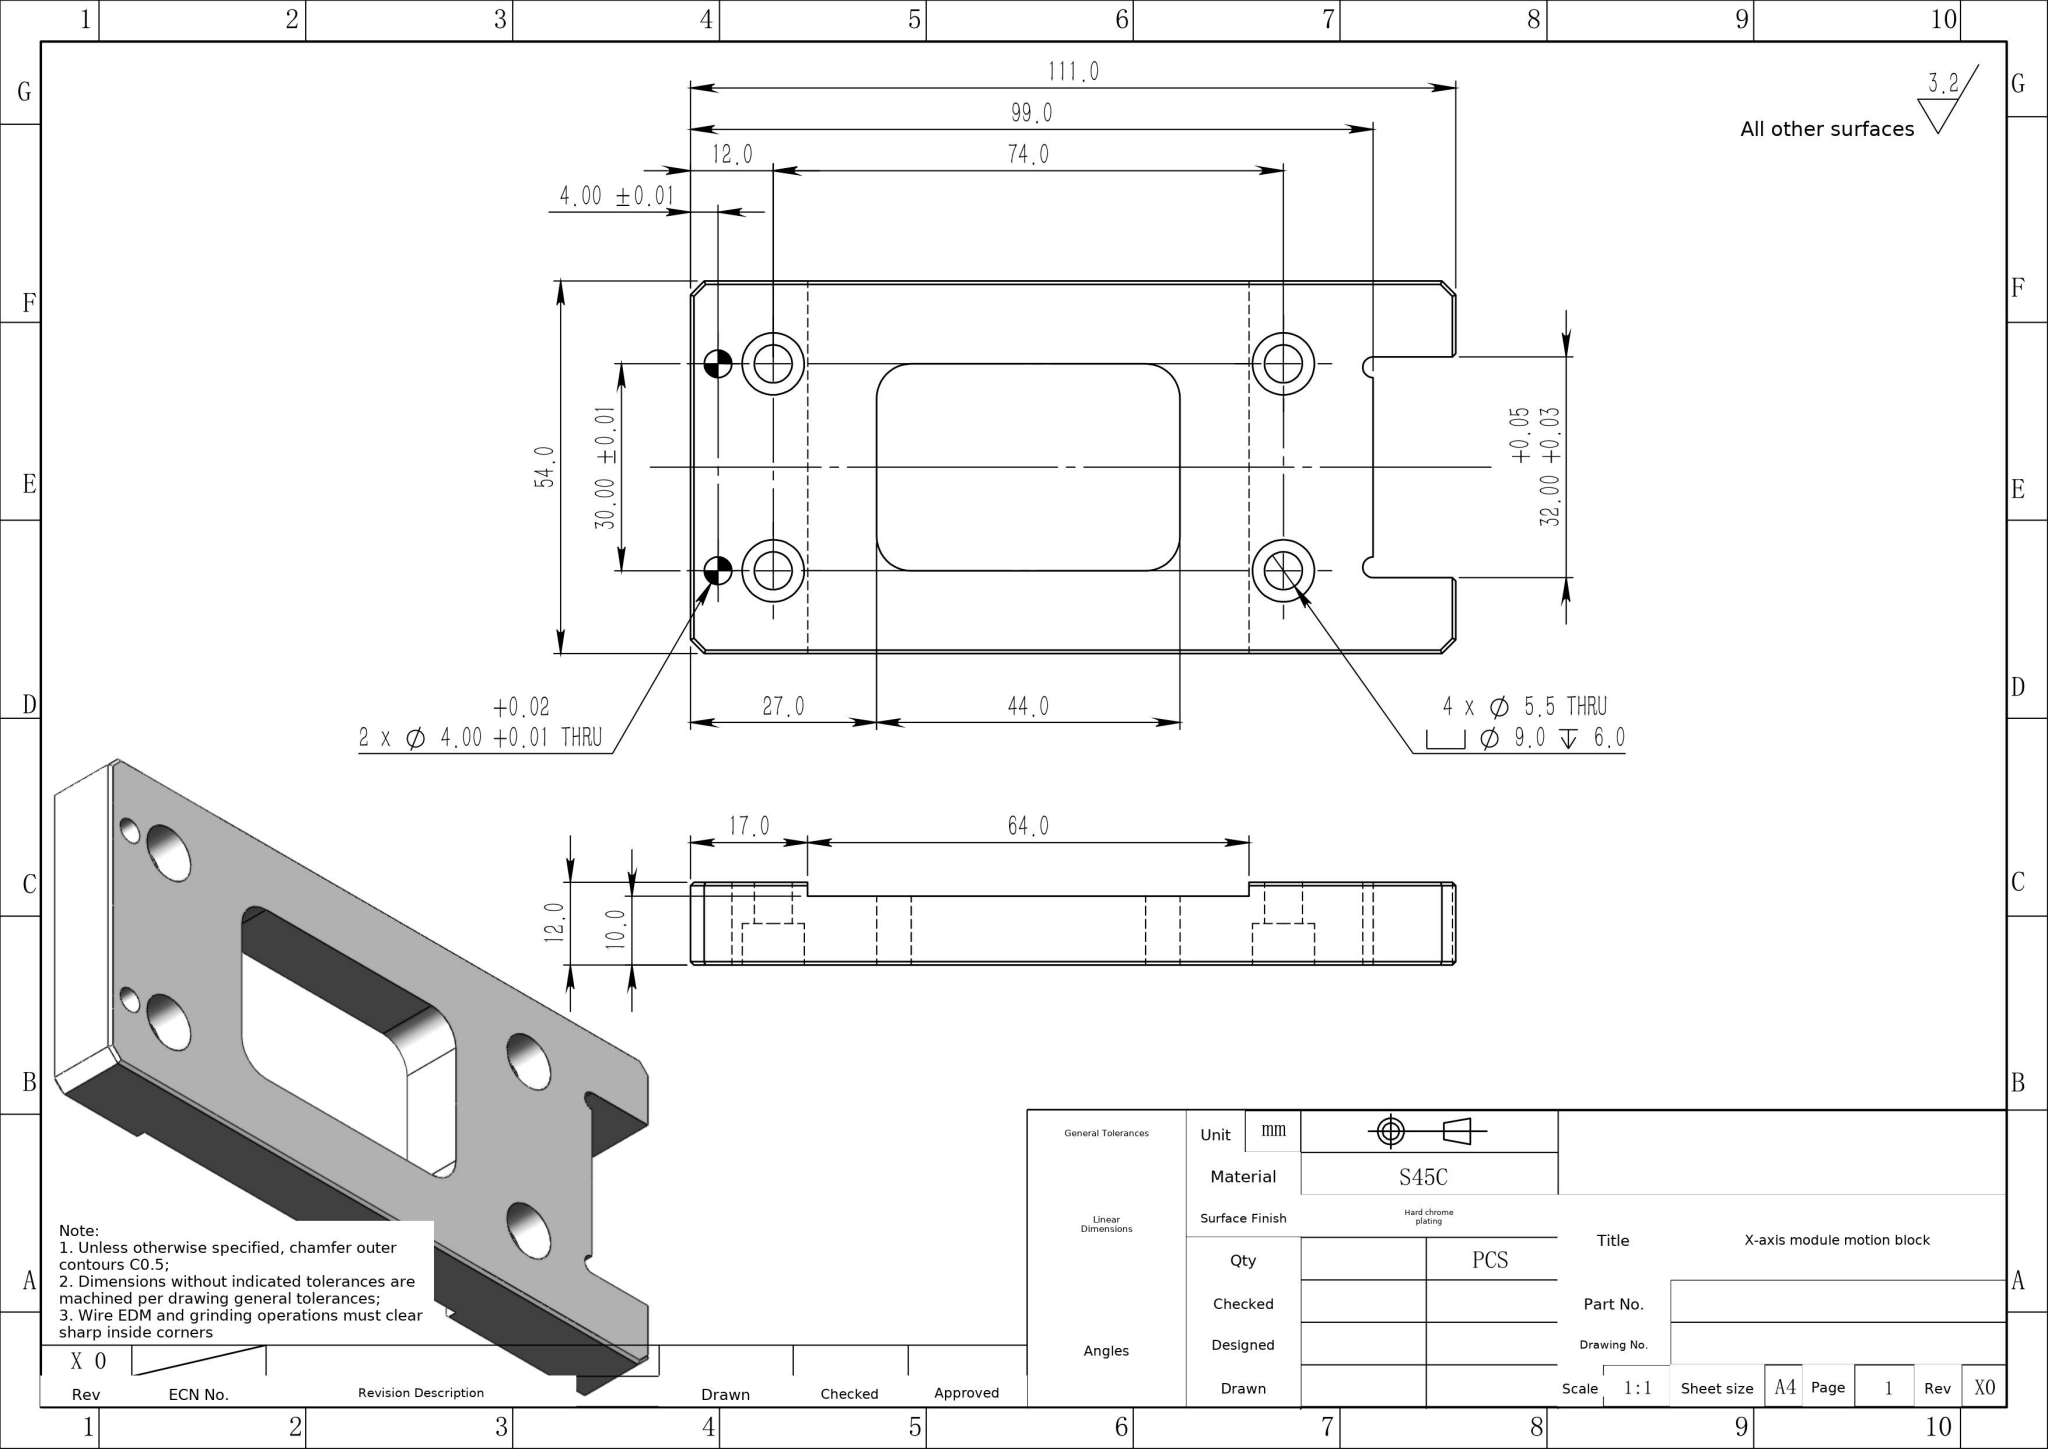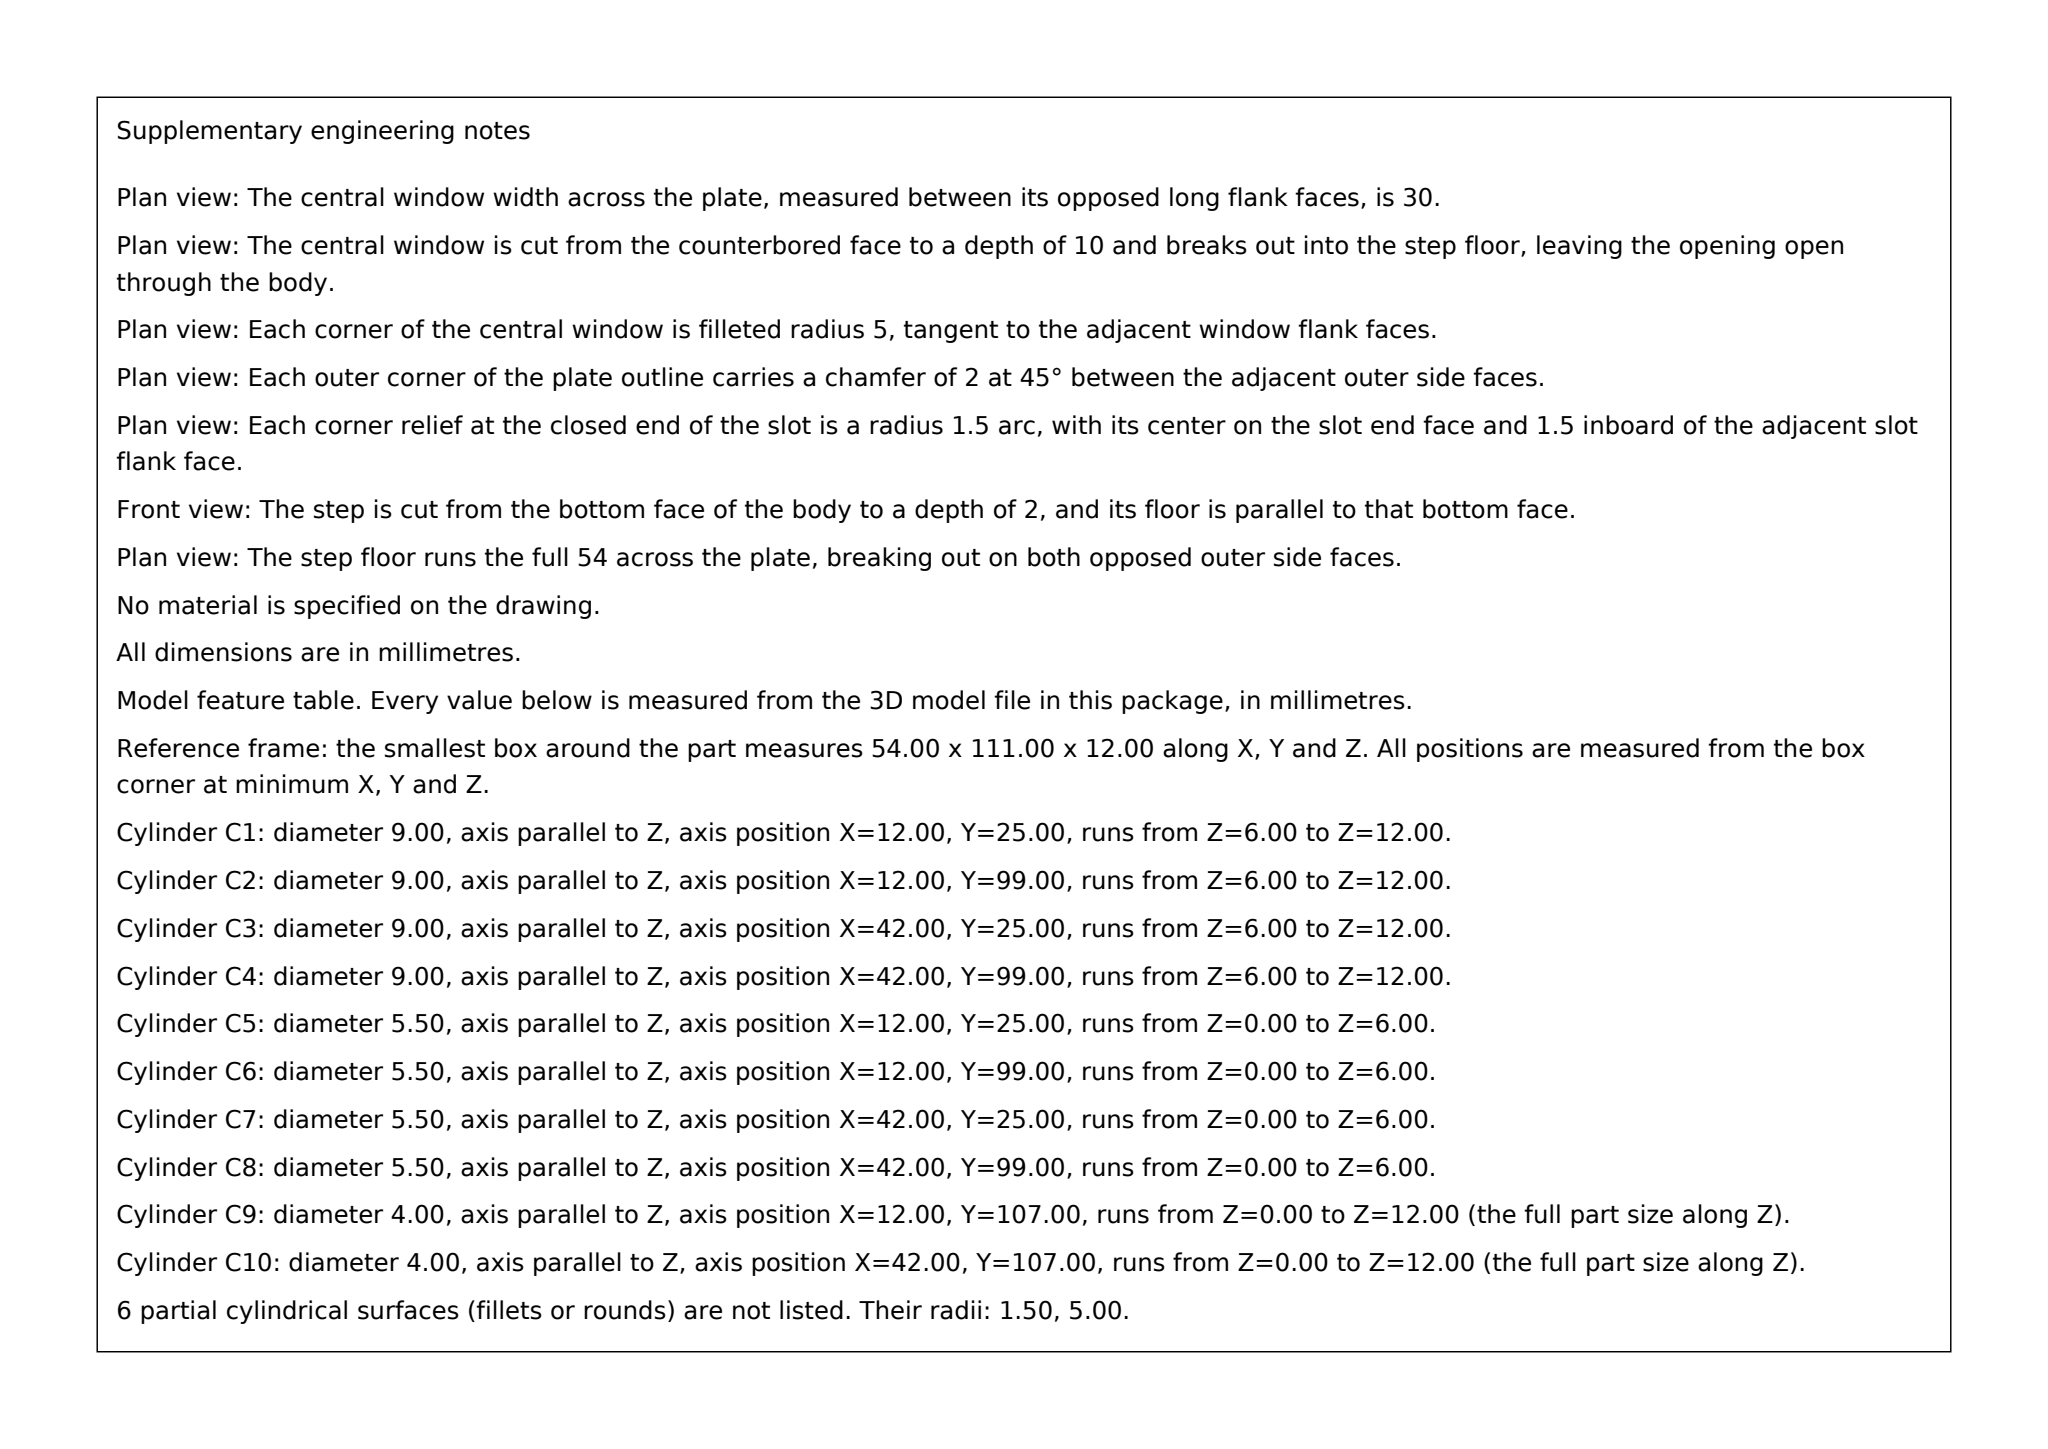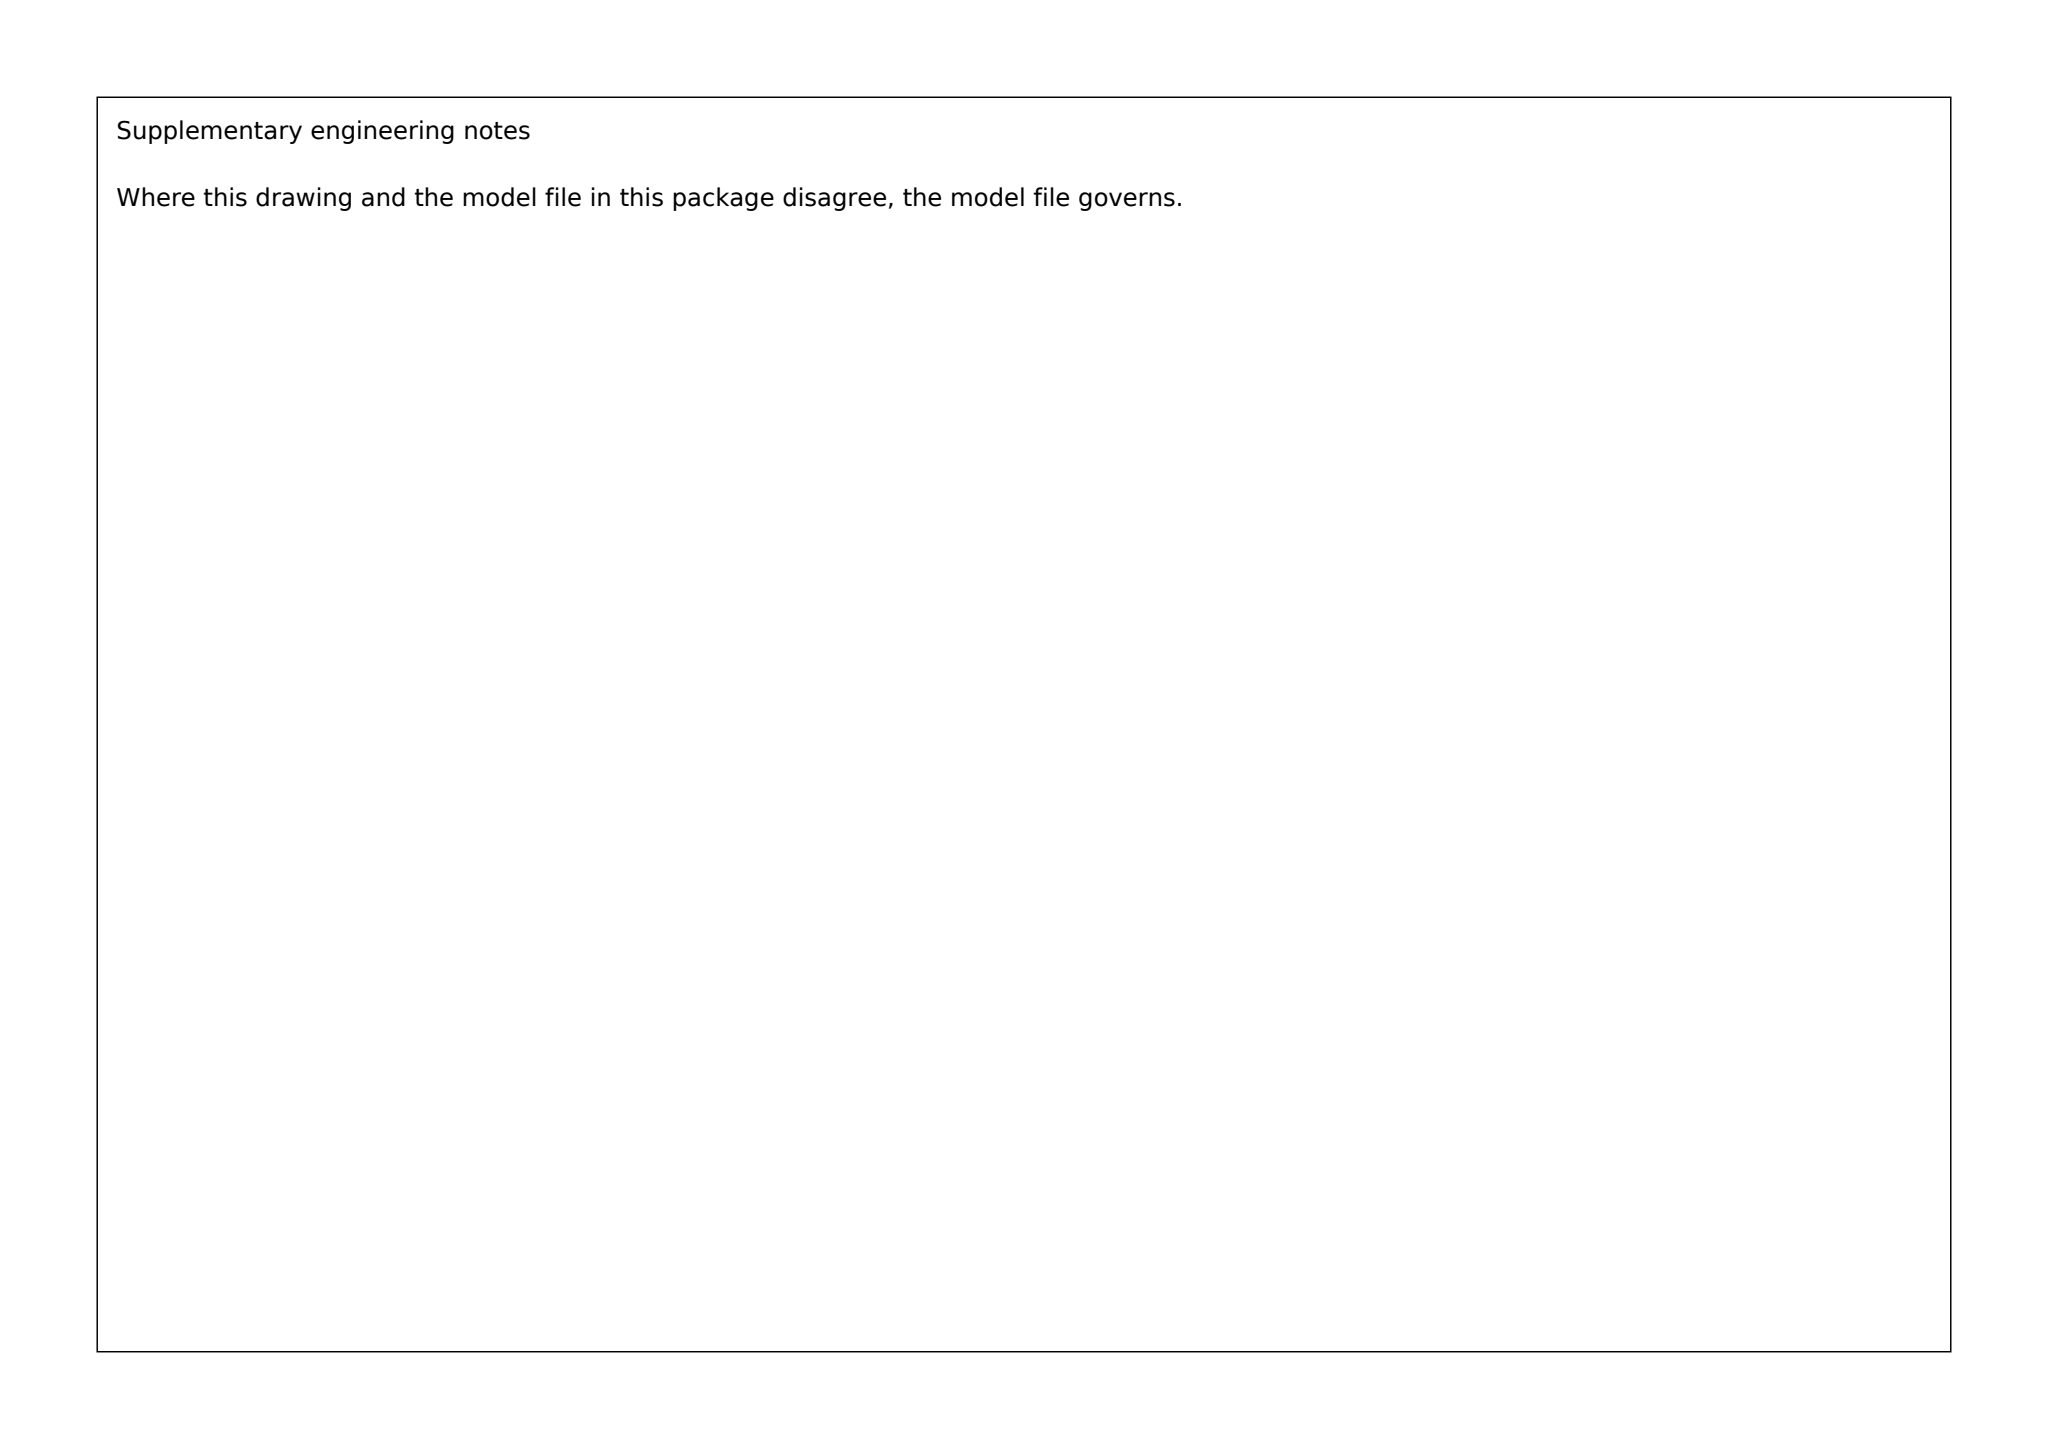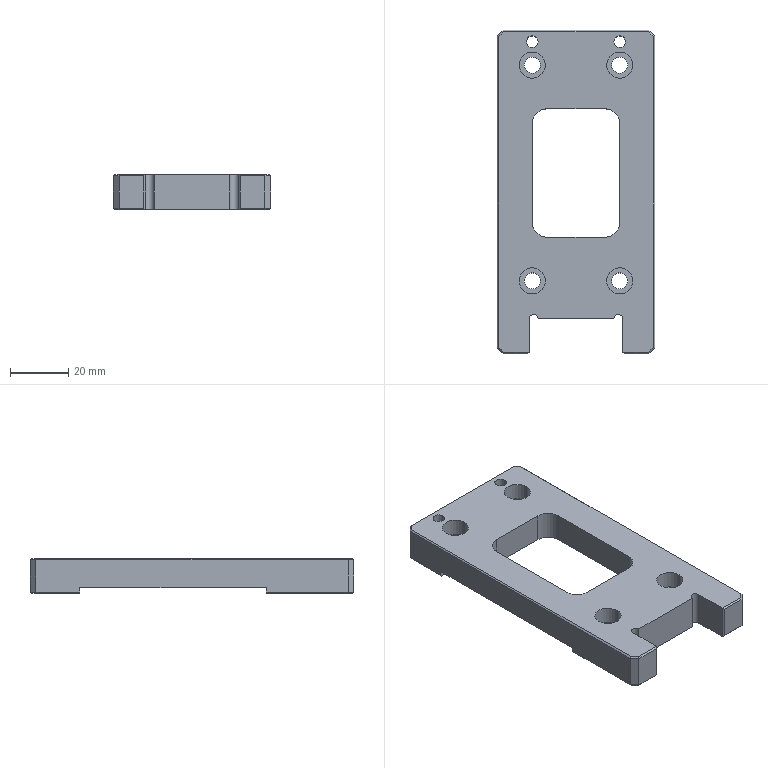Part | SolidWorks | mm | 1 solid | 74 faces | box 54 x 111 x 12 mm | volume 44783 mm3 | plane 48 | cylinder 26 | commonest cylinder face diameters 9 x8 5.5 x8 4 x4 10 x4 3 x2
build123d program:
from build123d import *

# Parameters (mm, degrees)
SKETCH1_W                                       = 54
SKETCH1_H                                       = 111
BOSS_EXTRUDE1_DEPTH                             = 12
M5_HEX_SOCKET_HEAD_CAP_SCREW_CBORE1_D           = 5.5
M5_HEX_SOCKET_HEAD_CAP_SCREW_CBORE1_CBORE_D     = 9
M5_HEX_SOCKET_HEAD_CAP_SCREW_CBORE1_CBORE_DEPTH = 6
SKETCH5_W                                       = 32
SKETCH5_H                                       = 12
CUT_EXTRUDE2_DEPTH                              = 63.875
SIZE_MM_DOWEL_PIN_HOLE1_D                       = 4
SKETCH8_R                                       = 1.5
CUT_EXTRUDE3_DEPTH                              = 63.875
SKETCH9_W                                       = 54
SKETCH9_H                                       = 64
CUT_EXTRUDE4_DEPTH                              = 2
SKETCH11_W                                      = 30
SKETCH11_H                                      = 44
CUT_EXTRUDE5_DEPTH                              = 63.524
CHAMFER1_SIZE                                   = 2
CHAMFER2_SIZE                                   = 0.5
FILLET1_R                                       = 5


with BuildPart() as part:
    # Sketch1 → Boss-Extrude1 (new body)
    with BuildSketch(Plane.XY):
        Rectangle(SKETCH1_W, SKETCH1_H)
    extrude(amount=-BOSS_EXTRUDE1_DEPTH)

    # M5 Hex Socket Head Cap Screw CBORE1 (through all)
    with Locations(Plane.XY):
        with Locations((-15, -30.5), (-15, 43.5), (15, 43.5), (15, -30.5)):
            CounterBoreHole(M5_HEX_SOCKET_HEAD_CAP_SCREW_CBORE1_D / 2, M5_HEX_SOCKET_HEAD_CAP_SCREW_CBORE1_CBORE_D / 2, M5_HEX_SOCKET_HEAD_CAP_SCREW_CBORE1_CBORE_DEPTH)

    # Sketch5 → Cut-Extrude2 (cut, through all)
    with BuildSketch(Plane.XY):
        with Locations((0, -49.5)):
            Rectangle(SKETCH5_W, SKETCH5_H)
    extrude(amount=-CUT_EXTRUDE2_DEPTH, mode=Mode.SUBTRACT)

    # Size mm Dowel Pin Hole1 (through all)
    with Locations(Plane.XY):
        with Locations((-15, 51.5), (15, 51.5)):
            Hole(SIZE_MM_DOWEL_PIN_HOLE1_D / 2)

    # Sketch8 → Cut-Extrude3 (cut, through all)
    with BuildSketch(Plane.XY):
        with Locations((-14.5, -43.5)):
            Circle(SKETCH8_R)
        with Locations((14.5, -43.5)):
            Circle(SKETCH8_R)
    extrude(amount=-CUT_EXTRUDE3_DEPTH, mode=Mode.SUBTRACT)

    # Sketch9 → Cut-Extrude4 (cut)
    with BuildSketch(Plane(origin=(0, 0, -12), x_dir=(-1, 0, 0), z_dir=(0, 0, -1))):
        with Locations((0, 6.5)):
            Rectangle(SKETCH9_W, SKETCH9_H)
    extrude(amount=-CUT_EXTRUDE4_DEPTH, mode=Mode.SUBTRACT)

    # Sketch11 → Cut-Extrude5 (cut, through all)
    with BuildSketch(Plane(origin=(0, 0, -10), x_dir=(-1, 0, 0), z_dir=(0, 0, -1))):
        with Locations((0, 6.5)):
            Rectangle(SKETCH11_W, SKETCH11_H)
    extrude(amount=-CUT_EXTRUDE5_DEPTH, mode=Mode.SUBTRACT)

    # Chamfer1
    chamfer1_edges = [part.edges().sort_by_distance(p)[0] for p in [
        (27, -55.5, -6),
        (-27, -55.5, -6),
        (-27, 55.5, -6),
        (27, 55.5, -6),
    ]]
    chamfer(chamfer1_edges, length=CHAMFER1_SIZE)

    # Chamfer2
    chamfer2_edges = [part.edges().sort_by_distance(p)[0] for p in [
        (27, 0, 0),
        (27, -39.5, -12),
        (0, 55.5, 0),
        (-27, 0, 0),
        (-20.5, -55.5, 0),
        (26, -54.5, 0),
        (-26, -54.5, 0),
        (-26, 54.5, 0),
        (26, 54.5, 0),
        (0, 55.5, -12),
        (-27, 46, -12),
        (-26, 54.5, -12),
        (26, 54.5, -12),
        (-20.5, -55.5, -12),
        (26, -54.5, -12),
        (-26, -54.5, -12),
        (20.5, -55.5, 0),
        (20.5, -55.5, -12),
        (-16, -55.5, -6),
        (16, -55.5, -6),
        (-27, -39.5, -12),
        (27, 46, -12),
    ]]
    chamfer(chamfer2_edges, length=CHAMFER2_SIZE)

    # Fillet1
    fillet1_edges = [part.edges().sort_by_distance(p)[0] for p in [
        (15, -15.5, -5),
        (15, 28.5, -5),
        (-15, 28.5, -5),
        (-15, -15.5, -5),
    ]]
    fillet(fillet1_edges, radius=FILLET1_R)


solid = part.part